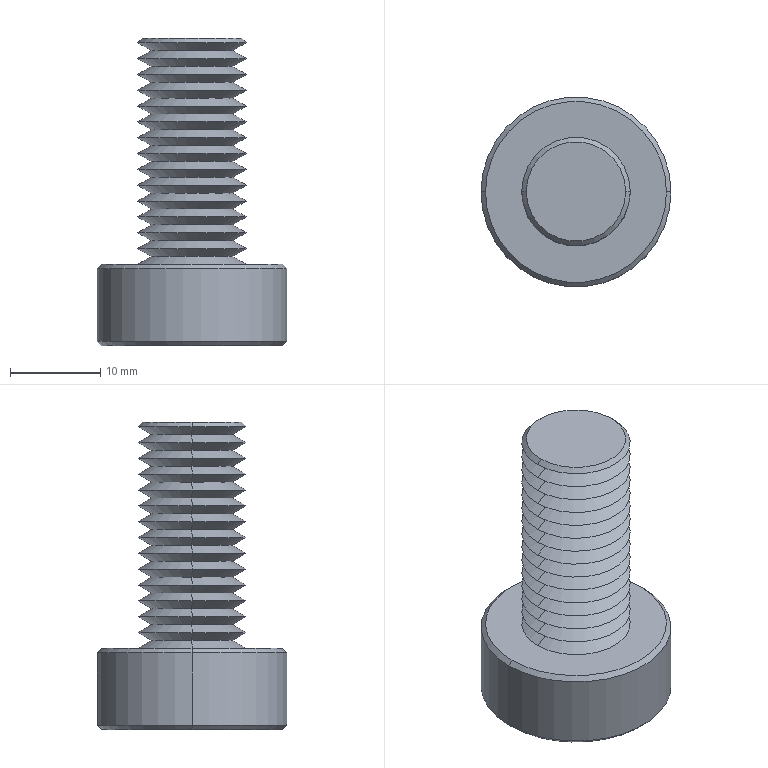Component | SolidWorks | M12LiftingEyeAssembly1-2_M12LiftingEyeInterruption-2 | 1 solid | 67 faces | box 21 x 21 x 34 mm | volume 5283 mm3 | cone 62 | plane 3 | cylinder 2 | commonest cylinder face diameters 21 x2
build123d program:
from build123d import *

# Parameters (mm, degrees)
LPATTERN1_COUNT = 14
LPATTERN1_PITCH = 1.75
CHAMFER1_SIZE   = 0.5


with BuildPart() as part:
    # Sketch18 → Revolve2 (revolve)
    with BuildSketch(Plane(origin=(0, 0, 0), x_dir=(0, 0, -1), z_dir=(1, 0, 0)), mode=Mode.PRIVATE) as revolve2_sk:
        Polygon((-50.931, 27.579), (-41.931, 27.579), (-41.931, 23.079), (-17.431, 23.079), (-16.931, 22.579), (-16.931, 17.079), (-50.931, 17.079), align=None)
    revolve(revolve2_sk.sketch.rotate(Axis((0, 17.079, 50.931), (0, 0, -1)), 90), axis=Axis((0, 17.079, 50.931), (0, 0, -1)))

    # Sketch19 → Cut-Revolve20 (revolve, cut)
    with BuildSketch(Plane(origin=(0, 0, 0), x_dir=(0, 0, -1), z_dir=(1, 0, 0)), mode=Mode.PRIVATE) as cut_revolve20_sk:
        Polygon((-17.431, 23.079), (-18.306, 21.564), (-19.181, 23.079), align=None)
    cut_revolve20 = revolve(cut_revolve20_sk.sketch.rotate(Axis((0, 17.079, 16.931), (0, 0, 1)), 90), axis=Axis((0, 17.079, 16.931), (0, 0, 1)), mode=Mode.SUBTRACT)

    # LPattern1: Cut-Revolve20 ×14
    with Locations(*[(0, 0, i * LPATTERN1_PITCH) for i in range(1, LPATTERN1_COUNT)]):
        add(cut_revolve20, mode=Mode.SUBTRACT)

    # Chamfer1
    chamfer1_edges = [part.edges().sort_by_distance(p)[0] for p in [
        (-10.5, 17.079, 41.931),
        (-10.5, 17.079, 50.931),
    ]]
    chamfer(chamfer1_edges, length=CHAMFER1_SIZE)


solid = part.part

# Placed as in the assembly
solid = solid.moved(Location((529.524, 14.342, 41.82), (180, 0, 0)))